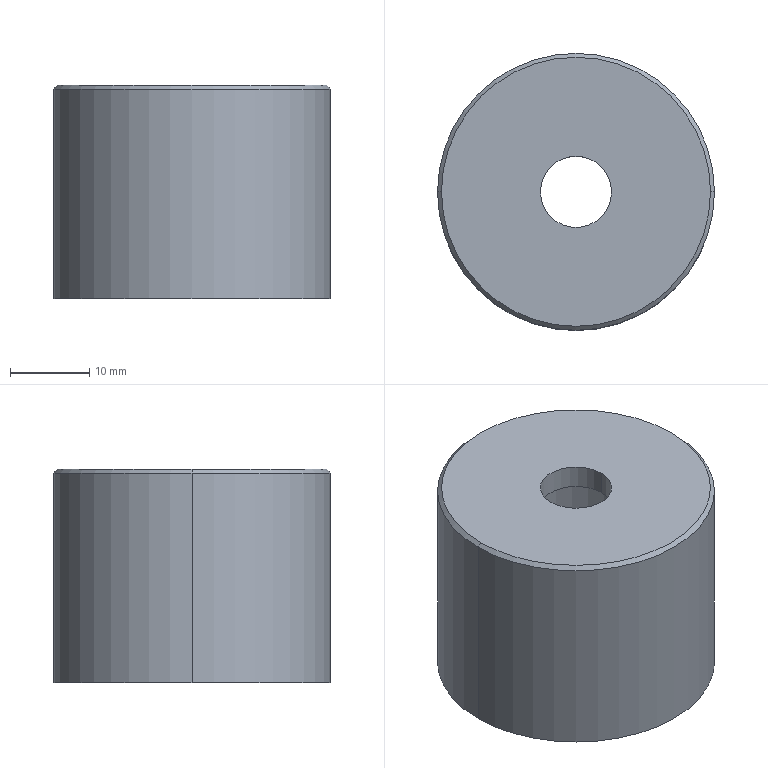Component | SolidWorks | YC1-250-03-01SliderAssembly-1_YC1-200-03-39SmallSprocketGland-1 | 1 solid | 11 faces | box 35 x 35 x 27 mm | volume 18233 mm3 | cylinder 6 | plane 3 | cone 2 | commonest cylinder face diameters 20 x2 35 x2 9 x2 | material Plain Carbon Steel
STEP:
#1=COLOUR_RGB('',0.7922,0.8196,0.9333);
#2=FILL_AREA_STYLE_COLOUR('',#1);
#3=FILL_AREA_STYLE('',(#2));
#4=SURFACE_STYLE_FILL_AREA(#3);
#5=SURFACE_SIDE_STYLE('',(#4));
#6=SURFACE_STYLE_USAGE(.BOTH.,#5);
#7=PRESENTATION_STYLE_ASSIGNMENT((#6));
#8=CARTESIAN_POINT('',(7.48,68.998,-11.339));
#9=VERTEX_POINT('',#8);
#10=CARTESIAN_POINT('',(6.693,68.998,-11.339));
#11=VERTEX_POINT('',#10);
#12=CARTESIAN_POINT('',(7.087,68.998,-11.339));
#13=DIRECTION('',(0.,0.,-1.));
#14=DIRECTION('',(-1.,0.,0.));
#15=AXIS2_PLACEMENT_3D('',#12,#13,#14);
#16=CIRCLE('',#15,0.3937);
#17=EDGE_CURVE('',#9,#11,#16,.T.);
#18=ORIENTED_EDGE('',*,*,#17,.F.);
#19=CARTESIAN_POINT('',(7.48,68.998,-12.283));
#20=VERTEX_POINT('',#19);
#21=CARTESIAN_POINT('',(7.48,68.998,-12.795));
#22=DIRECTION('',(0.,0.,-1.));
#23=VECTOR('',#22,39.37);
#24=LINE('',#21,#23);
#25=EDGE_CURVE('',#9,#20,#24,.T.);
#26=ORIENTED_EDGE('',*,*,#25,.T.);
#27=CARTESIAN_POINT('',(6.693,68.998,-12.283));
#28=VERTEX_POINT('',#27);
#29=CARTESIAN_POINT('',(7.087,68.998,-12.283));
#30=DIRECTION('',(0.,0.,1.));
#31=DIRECTION('',(1.,0.,0.));
#32=AXIS2_PLACEMENT_3D('',#29,#30,#31);
#33=CIRCLE('',#32,0.3937);
#34=EDGE_CURVE('',#28,#20,#33,.T.);
#35=ORIENTED_EDGE('',*,*,#34,.F.);
#36=CARTESIAN_POINT('',(6.693,68.998,-12.795));
#37=DIRECTION('',(0.,0.,-1.));
#38=VECTOR('',#37,39.37);
#39=LINE('',#36,#38);
#40=EDGE_CURVE('',#11,#28,#39,.T.);
#41=ORIENTED_EDGE('',*,*,#40,.F.);
#42=EDGE_LOOP('',(#18,#26,#35,#41));
#43=FACE_OUTER_BOUND('',#42,.T.);
#44=CARTESIAN_POINT('',(7.087,68.998,-12.795));
#45=DIRECTION('',(0.,0.,-1.));
#46=DIRECTION('',(-1.,0.,0.));
#47=AXIS2_PLACEMENT_3D('',#44,#45,#46);
#48=CYLINDRICAL_SURFACE('',#47,0.3937);
#49=ADVANCED_FACE('',(#43),#48,.F.);
#50=CARTESIAN_POINT('',(7.776,68.998,-12.283));
#51=VERTEX_POINT('',#50);
#52=CARTESIAN_POINT('',(6.398,68.998,-12.283));
#53=VERTEX_POINT('',#52);
#54=CARTESIAN_POINT('',(7.087,68.998,-12.283));
#55=DIRECTION('',(0.,0.,1.));
#56=DIRECTION('',(1.,0.,0.));
#57=AXIS2_PLACEMENT_3D('',#54,#55,#56);
#58=CIRCLE('',#57,0.689);
#59=EDGE_CURVE('',#51,#53,#58,.T.);
#60=ORIENTED_EDGE('',*,*,#59,.T.);
#61=CARTESIAN_POINT('',(6.398,68.998,-11.24));
#62=VERTEX_POINT('',#61);
#63=CARTESIAN_POINT('',(6.398,68.998,-11.22));
#64=DIRECTION('',(0.,0.,1.));
#65=VECTOR('',#64,39.37);
#66=LINE('',#63,#65);
#67=EDGE_CURVE('',#53,#62,#66,.T.);
#68=ORIENTED_EDGE('',*,*,#67,.T.);
#69=CARTESIAN_POINT('',(7.776,68.998,-11.24));
#70=VERTEX_POINT('',#69);
#71=CARTESIAN_POINT('',(7.087,68.998,-11.24));
#72=DIRECTION('',(0.,0.,-1.));
#73=DIRECTION('',(1.,0.,0.));
#74=AXIS2_PLACEMENT_3D('',#71,#72,#73);
#75=CIRCLE('',#74,0.689);
#76=EDGE_CURVE('',#62,#70,#75,.T.);
#77=ORIENTED_EDGE('',*,*,#76,.T.);
#78=CARTESIAN_POINT('',(7.776,68.998,-11.22));
#79=DIRECTION('',(0.,0.,1.));
#80=VECTOR('',#79,39.37);
#81=LINE('',#78,#80);
#82=EDGE_CURVE('',#51,#70,#81,.T.);
#83=ORIENTED_EDGE('',*,*,#82,.F.);
#84=EDGE_LOOP('',(#60,#68,#77,#83));
#85=FACE_OUTER_BOUND('',#84,.T.);
#86=CARTESIAN_POINT('',(7.087,68.998,-11.22));
#87=DIRECTION('',(0.,0.,1.));
#88=DIRECTION('',(1.,0.,0.));
#89=AXIS2_PLACEMENT_3D('',#86,#87,#88);
#90=CYLINDRICAL_SURFACE('',#89,0.689);
#91=ADVANCED_FACE('',(#85),#90,.T.);
#92=CARTESIAN_POINT('',(6.417,68.998,-11.22));
#93=VERTEX_POINT('',#92);
#94=CARTESIAN_POINT('',(7.756,68.998,-11.22));
#95=VERTEX_POINT('',#94);
#96=CARTESIAN_POINT('',(7.087,68.998,-11.22));
#97=DIRECTION('',(0.,0.,-1.));
#98=DIRECTION('',(-1.,0.,0.));
#99=AXIS2_PLACEMENT_3D('',#96,#97,#98);
#100=CIRCLE('',#99,0.6693);
#101=EDGE_CURVE('',#93,#95,#100,.T.);
#102=ORIENTED_EDGE('',*,*,#101,.T.);
#103=CARTESIAN_POINT('',(7.776,68.998,-11.24));
#104=DIRECTION('',(0.7071,0.,-0.7071));
#105=VECTOR('',#104,39.37);
#106=LINE('',#103,#105);
#107=EDGE_CURVE('',#95,#70,#106,.T.);
#108=ORIENTED_EDGE('',*,*,#107,.T.);
#109=ORIENTED_EDGE('',*,*,#76,.F.);
#110=CARTESIAN_POINT('',(6.398,68.998,-11.24));
#111=DIRECTION('',(-0.7071,0.,-0.7071));
#112=VECTOR('',#111,39.37);
#113=LINE('',#110,#112);
#114=EDGE_CURVE('',#93,#62,#113,.T.);
#115=ORIENTED_EDGE('',*,*,#114,.F.);
#116=EDGE_LOOP('',(#102,#108,#109,#115));
#117=FACE_OUTER_BOUND('',#116,.T.);
#118=CARTESIAN_POINT('',(7.087,68.998,-11.24));
#119=DIRECTION('',(0.,0.,-1.));
#120=DIRECTION('',(-1.,0.,0.));
#121=AXIS2_PLACEMENT_3D('',#118,#119,#120);
#122=CONICAL_SURFACE('',#121,0.689,0.7854);
#123=ADVANCED_FACE('',(#117),#122,.T.);
#124=CARTESIAN_POINT('',(6.909,68.998,-11.339));
#125=VERTEX_POINT('',#124);
#126=CARTESIAN_POINT('',(7.264,68.998,-11.339));
#127=VERTEX_POINT('',#126);
#128=CARTESIAN_POINT('',(7.087,68.998,-11.339));
#129=DIRECTION('',(0.,0.,1.));
#130=DIRECTION('',(1.,0.,0.));
#131=AXIS2_PLACEMENT_3D('',#128,#129,#130);
#132=CIRCLE('',#131,0.1772);
#133=EDGE_CURVE('',#125,#127,#132,.T.);
#134=ORIENTED_EDGE('',*,*,#133,.F.);
#135=CARTESIAN_POINT('',(6.909,68.998,-11.22));
#136=VERTEX_POINT('',#135);
#137=CARTESIAN_POINT('',(6.909,68.998,-11.22));
#138=DIRECTION('',(0.,0.,1.));
#139=VECTOR('',#138,39.37);
#140=LINE('',#137,#139);
#141=EDGE_CURVE('',#125,#136,#140,.T.);
#142=ORIENTED_EDGE('',*,*,#141,.T.);
#143=CARTESIAN_POINT('',(7.264,68.998,-11.22));
#144=VERTEX_POINT('',#143);
#145=CARTESIAN_POINT('',(7.087,68.998,-11.22));
#146=DIRECTION('',(0.,0.,1.));
#147=DIRECTION('',(1.,0.,0.));
#148=AXIS2_PLACEMENT_3D('',#145,#146,#147);
#149=CIRCLE('',#148,0.1772);
#150=EDGE_CURVE('',#136,#144,#149,.T.);
#151=ORIENTED_EDGE('',*,*,#150,.T.);
#152=CARTESIAN_POINT('',(7.264,68.998,-11.22));
#153=DIRECTION('',(0.,0.,1.));
#154=VECTOR('',#153,39.37);
#155=LINE('',#152,#154);
#156=EDGE_CURVE('',#127,#144,#155,.T.);
#157=ORIENTED_EDGE('',*,*,#156,.F.);
#158=EDGE_LOOP('',(#134,#142,#151,#157));
#159=FACE_OUTER_BOUND('',#158,.T.);
#160=CARTESIAN_POINT('',(7.087,68.998,-11.22));
#161=DIRECTION('',(0.,0.,1.));
#162=DIRECTION('',(1.,0.,0.));
#163=AXIS2_PLACEMENT_3D('',#160,#161,#162);
#164=CYLINDRICAL_SURFACE('',#163,0.1772);
#165=ADVANCED_FACE('',(#159),#164,.F.);
#166=ORIENTED_EDGE('',*,*,#67,.F.);
#167=CARTESIAN_POINT('',(7.087,68.998,-12.283));
#168=DIRECTION('',(0.,0.,1.));
#169=DIRECTION('',(1.,0.,0.));
#170=AXIS2_PLACEMENT_3D('',#167,#168,#169);
#171=CIRCLE('',#170,0.689);
#172=EDGE_CURVE('',#53,#51,#171,.T.);
#173=ORIENTED_EDGE('',*,*,#172,.T.);
#174=ORIENTED_EDGE('',*,*,#82,.T.);
#175=CARTESIAN_POINT('',(7.087,68.998,-11.24));
#176=DIRECTION('',(0.,0.,-1.));
#177=DIRECTION('',(1.,0.,0.));
#178=AXIS2_PLACEMENT_3D('',#175,#176,#177);
#179=CIRCLE('',#178,0.689);
#180=EDGE_CURVE('',#70,#62,#179,.T.);
#181=ORIENTED_EDGE('',*,*,#180,.T.);
#182=EDGE_LOOP('',(#166,#173,#174,#181));
#183=FACE_OUTER_BOUND('',#182,.T.);
#184=CARTESIAN_POINT('',(7.087,68.998,-11.22));
#185=DIRECTION('',(0.,0.,1.));
#186=DIRECTION('',(1.,0.,0.));
#187=AXIS2_PLACEMENT_3D('',#184,#185,#186);
#188=CYLINDRICAL_SURFACE('',#187,0.689);
#189=ADVANCED_FACE('',(#183),#188,.T.);
#190=ORIENTED_EDGE('',*,*,#107,.F.);
#191=CARTESIAN_POINT('',(7.087,68.998,-11.22));
#192=DIRECTION('',(0.,0.,-1.));
#193=DIRECTION('',(-1.,0.,0.));
#194=AXIS2_PLACEMENT_3D('',#191,#192,#193);
#195=CIRCLE('',#194,0.6693);
#196=EDGE_CURVE('',#95,#93,#195,.T.);
#197=ORIENTED_EDGE('',*,*,#196,.T.);
#198=ORIENTED_EDGE('',*,*,#114,.T.);
#199=ORIENTED_EDGE('',*,*,#180,.F.);
#200=EDGE_LOOP('',(#190,#197,#198,#199));
#201=FACE_OUTER_BOUND('',#200,.T.);
#202=CARTESIAN_POINT('',(7.087,68.998,-11.24));
#203=DIRECTION('',(0.,0.,-1.));
#204=DIRECTION('',(-1.,0.,0.));
#205=AXIS2_PLACEMENT_3D('',#202,#203,#204);
#206=CONICAL_SURFACE('',#205,0.689,0.7854);
#207=ADVANCED_FACE('',(#201),#206,.T.);
#208=ORIENTED_EDGE('',*,*,#34,.T.);
#209=CARTESIAN_POINT('',(7.087,68.998,-12.283));
#210=DIRECTION('',(0.,0.,1.));
#211=DIRECTION('',(1.,0.,0.));
#212=AXIS2_PLACEMENT_3D('',#209,#210,#211);
#213=CIRCLE('',#212,0.3937);
#214=EDGE_CURVE('',#20,#28,#213,.T.);
#215=ORIENTED_EDGE('',*,*,#214,.T.);
#216=EDGE_LOOP('',(#208,#215));
#217=FACE_BOUND('',#216,.T.);
#218=ORIENTED_EDGE('',*,*,#59,.F.);
#219=ORIENTED_EDGE('',*,*,#172,.F.);
#220=EDGE_LOOP('',(#218,#219));
#221=FACE_OUTER_BOUND('',#220,.T.);
#222=CARTESIAN_POINT('',(7.087,69.687,-12.283));
#223=DIRECTION('',(0.,0.,1.));
#224=DIRECTION('',(1.,0.,0.));
#225=AXIS2_PLACEMENT_3D('',#222,#223,#224);
#226=PLANE('',#225);
#227=ADVANCED_FACE('',(#217,#221),#226,.F.);
#228=ORIENTED_EDGE('',*,*,#101,.F.);
#229=ORIENTED_EDGE('',*,*,#196,.F.);
#230=EDGE_LOOP('',(#228,#229));
#231=FACE_OUTER_BOUND('',#230,.T.);
#232=CARTESIAN_POINT('',(7.087,68.998,-11.22));
#233=DIRECTION('',(0.,0.,1.));
#234=DIRECTION('',(1.,0.,0.));
#235=AXIS2_PLACEMENT_3D('',#232,#233,#234);
#236=CIRCLE('',#235,0.1772);
#237=EDGE_CURVE('',#144,#136,#236,.T.);
#238=ORIENTED_EDGE('',*,*,#237,.F.);
#239=ORIENTED_EDGE('',*,*,#150,.F.);
#240=EDGE_LOOP('',(#238,#239));
#241=FACE_BOUND('',#240,.T.);
#242=CARTESIAN_POINT('',(7.087,68.998,-11.22));
#243=DIRECTION('',(0.,0.,-1.));
#244=DIRECTION('',(-1.,0.,0.));
#245=AXIS2_PLACEMENT_3D('',#242,#243,#244);
#246=PLANE('',#245);
#247=ADVANCED_FACE('',(#231,#241),#246,.F.);
#248=ORIENTED_EDGE('',*,*,#141,.F.);
#249=CARTESIAN_POINT('',(7.087,68.998,-11.339));
#250=DIRECTION('',(0.,0.,1.));
#251=DIRECTION('',(1.,0.,0.));
#252=AXIS2_PLACEMENT_3D('',#249,#250,#251);
#253=CIRCLE('',#252,0.1772);
#254=EDGE_CURVE('',#127,#125,#253,.T.);
#255=ORIENTED_EDGE('',*,*,#254,.F.);
#256=ORIENTED_EDGE('',*,*,#156,.T.);
#257=ORIENTED_EDGE('',*,*,#237,.T.);
#258=EDGE_LOOP('',(#248,#255,#256,#257));
#259=FACE_OUTER_BOUND('',#258,.T.);
#260=CARTESIAN_POINT('',(7.087,68.998,-11.22));
#261=DIRECTION('',(0.,0.,1.));
#262=DIRECTION('',(1.,0.,0.));
#263=AXIS2_PLACEMENT_3D('',#260,#261,#262);
#264=CYLINDRICAL_SURFACE('',#263,0.1772);
#265=ADVANCED_FACE('',(#259),#264,.F.);
#266=ORIENTED_EDGE('',*,*,#254,.T.);
#267=ORIENTED_EDGE('',*,*,#133,.T.);
#268=EDGE_LOOP('',(#266,#267));
#269=FACE_BOUND('',#268,.T.);
#270=CARTESIAN_POINT('',(7.087,68.998,-11.339));
#271=DIRECTION('',(0.,0.,-1.));
#272=DIRECTION('',(-1.,0.,0.));
#273=AXIS2_PLACEMENT_3D('',#270,#271,#272);
#274=CIRCLE('',#273,0.3937);
#275=EDGE_CURVE('',#11,#9,#274,.T.);
#276=ORIENTED_EDGE('',*,*,#275,.T.);
#277=ORIENTED_EDGE('',*,*,#17,.T.);
#278=EDGE_LOOP('',(#276,#277));
#279=FACE_OUTER_BOUND('',#278,.T.);
#280=CARTESIAN_POINT('',(7.087,69.313,-11.339));
#281=DIRECTION('',(0.,0.,1.));
#282=DIRECTION('',(1.,0.,0.));
#283=AXIS2_PLACEMENT_3D('',#280,#281,#282);
#284=PLANE('',#283);
#285=ADVANCED_FACE('',(#269,#279),#284,.F.);
#286=ORIENTED_EDGE('',*,*,#25,.F.);
#287=ORIENTED_EDGE('',*,*,#275,.F.);
#288=ORIENTED_EDGE('',*,*,#40,.T.);
#289=ORIENTED_EDGE('',*,*,#214,.F.);
#290=EDGE_LOOP('',(#286,#287,#288,#289));
#291=FACE_OUTER_BOUND('',#290,.T.);
#292=CARTESIAN_POINT('',(7.087,68.998,-12.795));
#293=DIRECTION('',(0.,0.,-1.));
#294=DIRECTION('',(-1.,0.,0.));
#295=AXIS2_PLACEMENT_3D('',#292,#293,#294);
#296=CYLINDRICAL_SURFACE('',#295,0.3937);
#297=ADVANCED_FACE('',(#291),#296,.F.);
#298=CLOSED_SHELL('',(#49,#91,#123,#165,#189,#207,#227,#247,#265,#285,#297));
#299=MANIFOLD_SOLID_BREP('',#298);
#300=STYLED_ITEM('',(#7),#299);
#301=(LENGTH_UNIT()NAMED_UNIT(*)SI_UNIT($,.METRE.));
#302=LENGTH_MEASURE_WITH_UNIT(LENGTH_MEASURE(0.0254),#301);
#303=DIMENSIONAL_EXPONENTS(1.,0.,0.,0.,0.,0.,0.);
#304=(CONVERSION_BASED_UNIT('',#302)LENGTH_UNIT()NAMED_UNIT(#303));
#305=UNCERTAINTY_MEASURE_WITH_UNIT(LENGTH_MEASURE(0.00001),#304,'','');
#306=(NAMED_UNIT(*)PLANE_ANGLE_UNIT()SI_UNIT($,.RADIAN.));
#307=(NAMED_UNIT(*)SI_UNIT($,.STERADIAN.)SOLID_ANGLE_UNIT());
#308=(GEOMETRIC_REPRESENTATION_CONTEXT(3)GLOBAL_UNCERTAINTY_ASSIGNED_CONTEXT((#305))GLOBAL_UNIT_ASSIGNED_CONTEXT((#304,#306,#307))REPRESENTATION_CONTEXT('',''));
#309=MECHANICAL_DESIGN_GEOMETRIC_PRESENTATION_REPRESENTATION('',(#300),#308);
#310=PRESENTATION_LAYER_ASSIGNMENT('','',(#300));
#311=CARTESIAN_POINT('',(0.,0.,0.));
#312=DIRECTION('',(0.,0.,1.));
#313=DIRECTION('',(1.,0.,0.));
#314=AXIS2_PLACEMENT_3D('',#311,#312,#313);
#315=(LENGTH_UNIT()NAMED_UNIT(*)SI_UNIT($,.METRE.));
#316=LENGTH_MEASURE_WITH_UNIT(LENGTH_MEASURE(0.0254),#315);
#317=DIMENSIONAL_EXPONENTS(1.,0.,0.,0.,0.,0.,0.);
#318=(CONVERSION_BASED_UNIT('',#316)LENGTH_UNIT()NAMED_UNIT(#317));
#319=UNCERTAINTY_MEASURE_WITH_UNIT(LENGTH_MEASURE(0.00001),#318,'','');
#320=(NAMED_UNIT(*)PLANE_ANGLE_UNIT()SI_UNIT($,.RADIAN.));
#321=(NAMED_UNIT(*)SI_UNIT($,.STERADIAN.)SOLID_ANGLE_UNIT());
#322=(GEOMETRIC_REPRESENTATION_CONTEXT(3)GLOBAL_UNCERTAINTY_ASSIGNED_CONTEXT((#319))GLOBAL_UNIT_ASSIGNED_CONTEXT((#318,#320,#321))REPRESENTATION_CONTEXT('',''));
#323=ADVANCED_BREP_SHAPE_REPRESENTATION('',(#299,#314),#322);